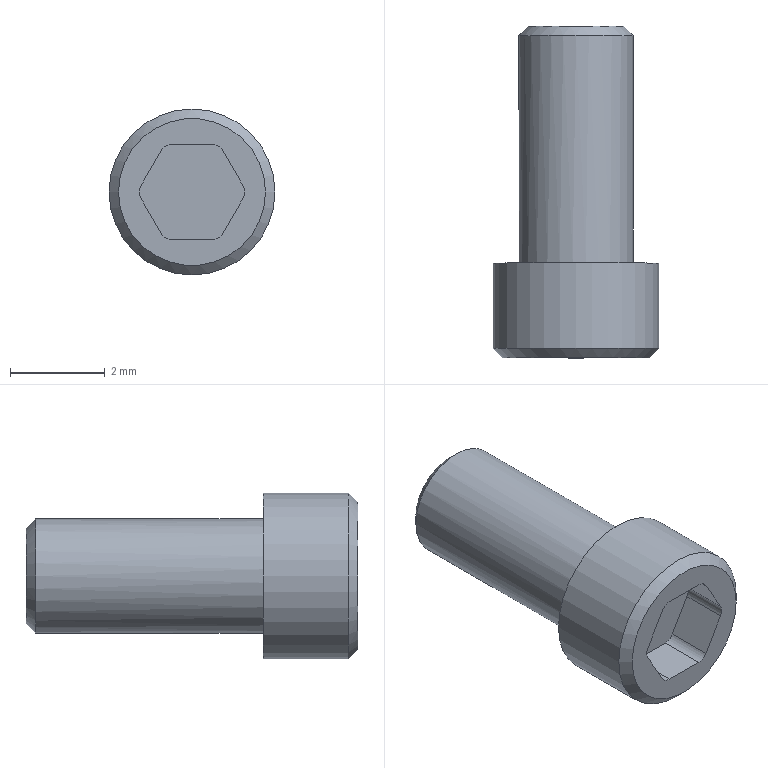Component | NX | SCREW_M2_5X5_2 | 1 solid | 20 faces | volume 38 mm3 | plane 10 | cylinder 8 | cone 2 | commonest cylinder face diameters 0.5 x6 2.41 x1 3.5 x1